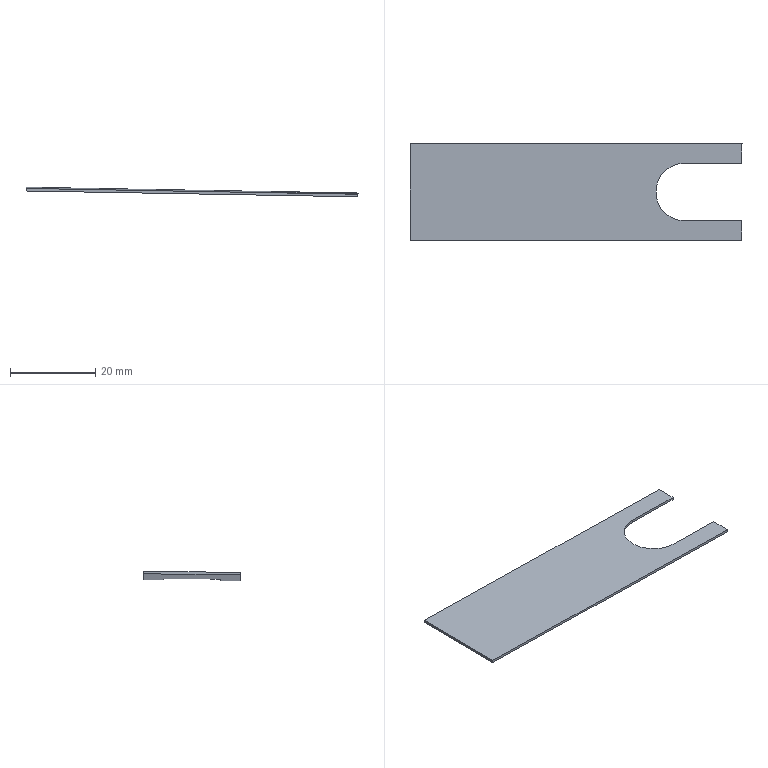Component | SolidWorks | 00-VacuumSuctionCupAssembly-1_02-TopCoverPlate-1 | 1 solid | 10 faces | box 78 x 22.66 x 2.25 mm | volume 908 mm3 | plane 9 | cylinder 1 | commonest cylinder face diameters 13.5 x1
build123d program:
from build123d import *

# Parameters (mm, degrees)
BOSS_EXTRUDE1_DEPTH = 2
SCALE1_SCALE        = 0.3


with BuildPart() as part:
    # Sketch1 → Boss-Extrude1 (new body)
    with BuildSketch(Plane(origin=(0, 2, 0), x_dir=(1, 0, 0), z_dir=(0, 1, 0))):
        with BuildLine():
            Line((45, -22.5), (0, -22.5))
            Line((0, -22.5), (0, -37.75))
            Line((0, -37.75), (260, -37.75))
            Line((260, -37.75), (260, 37.75))
            Line((260, 37.75), (0, 37.75))
            Line((0, 37.75), (0, 22.5))
            Line((0, 22.5), (45, 22.5))
            ThreePointArc((45, 22.5), (67.5, 0), (45, -22.5))
        make_face()
    extrude(amount=-BOSS_EXTRUDE1_DEPTH)


with BuildPart() as part_1:
    # Scale1: scaled about (146.519, 1, 0)
    add(part.part.scale(SCALE1_SCALE).moved(Location((102.564, 0.7, 0))))


solid = part_1.part

# Placed as in the assembly
solid = solid.moved(Location((174.24, 133.834, 29.789), (-89.279, 0.01259, -179)))
STEP:
#1=COLOUR_RGB('',0.7922,0.8196,0.9333);
#2=FILL_AREA_STYLE_COLOUR('',#1);
#3=FILL_AREA_STYLE('',(#2));
#4=SURFACE_STYLE_FILL_AREA(#3);
#5=SURFACE_SIDE_STYLE('',(#4));
#6=SURFACE_STYLE_USAGE(.BOTH.,#5);
#7=PRESENTATION_STYLE_ASSIGNMENT((#6));
#8=CARTESIAN_POINT('',(2.292,5.534,1.283));
#9=VERTEX_POINT('',#8);
#10=CARTESIAN_POINT('',(2.292,5.003,1.277));
#11=VERTEX_POINT('',#10);
#12=CARTESIAN_POINT('',(2.292,5.269,1.28));
#13=DIRECTION('',(0.01745,-0.01259,0.9998));
#14=DIRECTION('',(0.0002197,0.9999,0.01259));
#15=AXIS2_PLACEMENT_3D('',#12,#13,#14);
#16=CIRCLE('',#15,0.2657);
#17=EDGE_CURVE('',#9,#11,#16,.T.);
#18=ORIENTED_EDGE('',*,*,#17,.F.);
#19=CARTESIAN_POINT('',(2.292,5.534,1.307));
#20=VERTEX_POINT('',#19);
#21=CARTESIAN_POINT('',(2.292,5.534,1.307));
#22=DIRECTION('',(-0.01745,0.01259,-0.9998));
#23=VECTOR('',#22,39.37);
#24=LINE('',#21,#23);
#25=EDGE_CURVE('',#20,#9,#24,.T.);
#26=ORIENTED_EDGE('',*,*,#25,.F.);
#27=CARTESIAN_POINT('',(2.292,5.003,1.3));
#28=VERTEX_POINT('',#27);
#29=CARTESIAN_POINT('',(2.292,5.268,1.304));
#30=DIRECTION('',(0.01745,-0.01259,0.9998));
#31=DIRECTION('',(0.0002197,0.9999,0.01259));
#32=AXIS2_PLACEMENT_3D('',#29,#30,#31);
#33=CIRCLE('',#32,0.2657);
#34=EDGE_CURVE('',#20,#28,#33,.T.);
#35=ORIENTED_EDGE('',*,*,#34,.T.);
#36=CARTESIAN_POINT('',(2.292,5.003,1.3));
#37=DIRECTION('',(-0.01745,0.01259,-0.9998));
#38=VECTOR('',#37,39.37);
#39=LINE('',#36,#38);
#40=EDGE_CURVE('',#28,#11,#39,.T.);
#41=ORIENTED_EDGE('',*,*,#40,.T.);
#42=EDGE_LOOP('',(#18,#26,#35,#41));
#43=FACE_OUTER_BOUND('',#42,.T.);
#44=CARTESIAN_POINT('',(2.292,5.268,1.304));
#45=DIRECTION('',(-0.01745,0.01259,-0.9998));
#46=DIRECTION('',(-0.0002197,-0.9999,-0.01259));
#47=AXIS2_PLACEMENT_3D('',#44,#45,#46);
#48=CYLINDRICAL_SURFACE('',#47,0.2657);
#49=ADVANCED_FACE('',(#43),#48,.F.);
#50=CARTESIAN_POINT('',(2.823,5.534,1.274));
#51=VERTEX_POINT('',#50);
#52=CARTESIAN_POINT('',(2.823,5.534,1.274));
#53=DIRECTION('',(-0.9998,0.,0.01745));
#54=VECTOR('',#53,39.37);
#55=LINE('',#52,#54);
#56=EDGE_CURVE('',#51,#9,#55,.T.);
#57=ORIENTED_EDGE('',*,*,#56,.F.);
#58=CARTESIAN_POINT('',(2.823,5.534,1.298));
#59=VERTEX_POINT('',#58);
#60=CARTESIAN_POINT('',(2.823,5.534,1.298));
#61=DIRECTION('',(-0.01745,0.01259,-0.9998));
#62=VECTOR('',#61,39.37);
#63=LINE('',#60,#62);
#64=EDGE_CURVE('',#59,#51,#63,.T.);
#65=ORIENTED_EDGE('',*,*,#64,.F.);
#66=CARTESIAN_POINT('',(2.823,5.534,1.298));
#67=DIRECTION('',(-0.9998,0.,0.01745));
#68=VECTOR('',#67,39.37);
#69=LINE('',#66,#68);
#70=EDGE_CURVE('',#59,#20,#69,.T.);
#71=ORIENTED_EDGE('',*,*,#70,.T.);
#72=ORIENTED_EDGE('',*,*,#25,.T.);
#73=EDGE_LOOP('',(#57,#65,#71,#72));
#74=FACE_OUTER_BOUND('',#73,.T.);
#75=CARTESIAN_POINT('',(2.823,5.534,1.298));
#76=DIRECTION('',(-0.0002197,-0.9999,-0.01259));
#77=DIRECTION('',(-0.9998,0.,0.01745));
#78=AXIS2_PLACEMENT_3D('',#75,#76,#77);
#79=PLANE('',#78);
#80=ADVANCED_FACE('',(#74),#79,.T.);
#81=CARTESIAN_POINT('',(2.823,5.715,1.276));
#82=VERTEX_POINT('',#81);
#83=CARTESIAN_POINT('',(2.823,5.715,1.276));
#84=DIRECTION('',(-0.0002197,-0.9999,-0.01259));
#85=VECTOR('',#84,39.37);
#86=LINE('',#83,#85);
#87=EDGE_CURVE('',#82,#51,#86,.T.);
#88=ORIENTED_EDGE('',*,*,#87,.F.);
#89=CARTESIAN_POINT('',(2.824,5.714,1.3));
#90=VERTEX_POINT('',#89);
#91=CARTESIAN_POINT('',(2.824,5.714,1.3));
#92=DIRECTION('',(-0.01745,0.01259,-0.9998));
#93=VECTOR('',#92,39.37);
#94=LINE('',#91,#93);
#95=EDGE_CURVE('',#90,#82,#94,.T.);
#96=ORIENTED_EDGE('',*,*,#95,.F.);
#97=CARTESIAN_POINT('',(2.824,5.714,1.3));
#98=DIRECTION('',(-0.0002197,-0.9999,-0.01259));
#99=VECTOR('',#98,39.37);
#100=LINE('',#97,#99);
#101=EDGE_CURVE('',#90,#59,#100,.T.);
#102=ORIENTED_EDGE('',*,*,#101,.T.);
#103=ORIENTED_EDGE('',*,*,#64,.T.);
#104=EDGE_LOOP('',(#88,#96,#102,#103));
#105=FACE_OUTER_BOUND('',#104,.T.);
#106=CARTESIAN_POINT('',(2.824,5.714,1.3));
#107=DIRECTION('',(0.9998,-0.,-0.01745));
#108=DIRECTION('',(-0.0002197,-0.9999,-0.01259));
#109=AXIS2_PLACEMENT_3D('',#106,#107,#108);
#110=PLANE('',#109);
#111=ADVANCED_FACE('',(#105),#110,.T.);
#112=CARTESIAN_POINT('',(-0.2473,5.715,1.33));
#113=VERTEX_POINT('',#112);
#114=CARTESIAN_POINT('',(-0.2473,5.715,1.33));
#115=DIRECTION('',(0.9998,-0.,-0.01745));
#116=VECTOR('',#115,39.37);
#117=LINE('',#114,#116);
#118=EDGE_CURVE('',#113,#82,#117,.T.);
#119=ORIENTED_EDGE('',*,*,#118,.F.);
#120=CARTESIAN_POINT('',(-0.2469,5.714,1.354));
#121=VERTEX_POINT('',#120);
#122=CARTESIAN_POINT('',(-0.2469,5.714,1.354));
#123=DIRECTION('',(-0.01745,0.01259,-0.9998));
#124=VECTOR('',#123,39.37);
#125=LINE('',#122,#124);
#126=EDGE_CURVE('',#121,#113,#125,.T.);
#127=ORIENTED_EDGE('',*,*,#126,.F.);
#128=CARTESIAN_POINT('',(-0.2469,5.714,1.354));
#129=DIRECTION('',(0.9998,-0.,-0.01745));
#130=VECTOR('',#129,39.37);
#131=LINE('',#128,#130);
#132=EDGE_CURVE('',#121,#90,#131,.T.);
#133=ORIENTED_EDGE('',*,*,#132,.T.);
#134=ORIENTED_EDGE('',*,*,#95,.T.);
#135=EDGE_LOOP('',(#119,#127,#133,#134));
#136=FACE_OUTER_BOUND('',#135,.T.);
#137=CARTESIAN_POINT('',(-0.2469,5.714,1.354));
#138=DIRECTION('',(0.0002197,0.9999,0.01259));
#139=DIRECTION('',(0.9998,-0.,-0.01745));
#140=AXIS2_PLACEMENT_3D('',#137,#138,#139);
#141=PLANE('',#140);
#142=ADVANCED_FACE('',(#136),#141,.T.);
#143=CARTESIAN_POINT('',(-0.2475,4.823,1.319));
#144=VERTEX_POINT('',#143);
#145=CARTESIAN_POINT('',(-0.2475,4.823,1.319));
#146=DIRECTION('',(0.0002197,0.9999,0.01259));
#147=VECTOR('',#146,39.37);
#148=LINE('',#145,#147);
#149=EDGE_CURVE('',#144,#113,#148,.T.);
#150=ORIENTED_EDGE('',*,*,#149,.F.);
#151=CARTESIAN_POINT('',(-0.2471,4.823,1.342));
#152=VERTEX_POINT('',#151);
#153=CARTESIAN_POINT('',(-0.2471,4.823,1.342));
#154=DIRECTION('',(-0.01745,0.01259,-0.9998));
#155=VECTOR('',#154,39.37);
#156=LINE('',#153,#155);
#157=EDGE_CURVE('',#152,#144,#156,.T.);
#158=ORIENTED_EDGE('',*,*,#157,.F.);
#159=CARTESIAN_POINT('',(-0.2471,4.823,1.342));
#160=DIRECTION('',(0.0002197,0.9999,0.01259));
#161=VECTOR('',#160,39.37);
#162=LINE('',#159,#161);
#163=EDGE_CURVE('',#152,#121,#162,.T.);
#164=ORIENTED_EDGE('',*,*,#163,.T.);
#165=ORIENTED_EDGE('',*,*,#126,.T.);
#166=EDGE_LOOP('',(#150,#158,#164,#165));
#167=FACE_OUTER_BOUND('',#166,.T.);
#168=CARTESIAN_POINT('',(-0.2471,4.823,1.342));
#169=DIRECTION('',(-0.9998,0.,0.01745));
#170=DIRECTION('',(0.0002197,0.9999,0.01259));
#171=AXIS2_PLACEMENT_3D('',#168,#169,#170);
#172=PLANE('',#171);
#173=ADVANCED_FACE('',(#167),#172,.T.);
#174=CARTESIAN_POINT('',(2.823,4.823,1.265));
#175=VERTEX_POINT('',#174);
#176=CARTESIAN_POINT('',(2.823,4.823,1.265));
#177=DIRECTION('',(-0.9998,0.,0.01745));
#178=VECTOR('',#177,39.37);
#179=LINE('',#176,#178);
#180=EDGE_CURVE('',#175,#144,#179,.T.);
#181=ORIENTED_EDGE('',*,*,#180,.F.);
#182=CARTESIAN_POINT('',(2.823,4.823,1.289));
#183=VERTEX_POINT('',#182);
#184=CARTESIAN_POINT('',(2.823,4.823,1.289));
#185=DIRECTION('',(-0.01745,0.01259,-0.9998));
#186=VECTOR('',#185,39.37);
#187=LINE('',#184,#186);
#188=EDGE_CURVE('',#183,#175,#187,.T.);
#189=ORIENTED_EDGE('',*,*,#188,.F.);
#190=CARTESIAN_POINT('',(2.823,4.823,1.289));
#191=DIRECTION('',(-0.9998,0.,0.01745));
#192=VECTOR('',#191,39.37);
#193=LINE('',#190,#192);
#194=EDGE_CURVE('',#183,#152,#193,.T.);
#195=ORIENTED_EDGE('',*,*,#194,.T.);
#196=ORIENTED_EDGE('',*,*,#157,.T.);
#197=EDGE_LOOP('',(#181,#189,#195,#196));
#198=FACE_OUTER_BOUND('',#197,.T.);
#199=CARTESIAN_POINT('',(2.823,4.823,1.289));
#200=DIRECTION('',(-0.0002197,-0.9999,-0.01259));
#201=DIRECTION('',(-0.9998,0.,0.01745));
#202=AXIS2_PLACEMENT_3D('',#199,#200,#201);
#203=PLANE('',#202);
#204=ADVANCED_FACE('',(#198),#203,.T.);
#205=CARTESIAN_POINT('',(2.823,5.003,1.267));
#206=VERTEX_POINT('',#205);
#207=CARTESIAN_POINT('',(2.823,5.003,1.267));
#208=DIRECTION('',(-0.0002197,-0.9999,-0.01259));
#209=VECTOR('',#208,39.37);
#210=LINE('',#207,#209);
#211=EDGE_CURVE('',#206,#175,#210,.T.);
#212=ORIENTED_EDGE('',*,*,#211,.F.);
#213=CARTESIAN_POINT('',(2.823,5.003,1.291));
#214=VERTEX_POINT('',#213);
#215=CARTESIAN_POINT('',(2.823,5.003,1.291));
#216=DIRECTION('',(-0.01745,0.01259,-0.9998));
#217=VECTOR('',#216,39.37);
#218=LINE('',#215,#217);
#219=EDGE_CURVE('',#214,#206,#218,.T.);
#220=ORIENTED_EDGE('',*,*,#219,.F.);
#221=CARTESIAN_POINT('',(2.823,5.003,1.291));
#222=DIRECTION('',(-0.0002197,-0.9999,-0.01259));
#223=VECTOR('',#222,39.37);
#224=LINE('',#221,#223);
#225=EDGE_CURVE('',#214,#183,#224,.T.);
#226=ORIENTED_EDGE('',*,*,#225,.T.);
#227=ORIENTED_EDGE('',*,*,#188,.T.);
#228=EDGE_LOOP('',(#212,#220,#226,#227));
#229=FACE_OUTER_BOUND('',#228,.T.);
#230=CARTESIAN_POINT('',(2.823,5.003,1.291));
#231=DIRECTION('',(0.9998,-0.,-0.01745));
#232=DIRECTION('',(-0.0002197,-0.9999,-0.01259));
#233=AXIS2_PLACEMENT_3D('',#230,#231,#232);
#234=PLANE('',#233);
#235=ADVANCED_FACE('',(#229),#234,.T.);
#236=CARTESIAN_POINT('',(2.292,5.003,1.277));
#237=DIRECTION('',(0.9998,-0.,-0.01745));
#238=VECTOR('',#237,39.37);
#239=LINE('',#236,#238);
#240=EDGE_CURVE('',#11,#206,#239,.T.);
#241=ORIENTED_EDGE('',*,*,#240,.F.);
#242=ORIENTED_EDGE('',*,*,#40,.F.);
#243=CARTESIAN_POINT('',(2.292,5.003,1.3));
#244=DIRECTION('',(0.9998,-0.,-0.01745));
#245=VECTOR('',#244,39.37);
#246=LINE('',#243,#245);
#247=EDGE_CURVE('',#28,#214,#246,.T.);
#248=ORIENTED_EDGE('',*,*,#247,.T.);
#249=ORIENTED_EDGE('',*,*,#219,.T.);
#250=EDGE_LOOP('',(#241,#242,#248,#249));
#251=FACE_OUTER_BOUND('',#250,.T.);
#252=CARTESIAN_POINT('',(2.292,5.003,1.3));
#253=DIRECTION('',(0.0002197,0.9999,0.01259));
#254=DIRECTION('',(0.9998,-0.,-0.01745));
#255=AXIS2_PLACEMENT_3D('',#252,#253,#254);
#256=PLANE('',#255);
#257=ADVANCED_FACE('',(#251),#256,.T.);
#258=ORIENTED_EDGE('',*,*,#34,.F.);
#259=ORIENTED_EDGE('',*,*,#70,.F.);
#260=ORIENTED_EDGE('',*,*,#101,.F.);
#261=ORIENTED_EDGE('',*,*,#132,.F.);
#262=ORIENTED_EDGE('',*,*,#163,.F.);
#263=ORIENTED_EDGE('',*,*,#194,.F.);
#264=ORIENTED_EDGE('',*,*,#225,.F.);
#265=ORIENTED_EDGE('',*,*,#247,.F.);
#266=EDGE_LOOP('',(#258,#259,#260,#261,#262,#263,#264,#265));
#267=FACE_OUTER_BOUND('',#266,.T.);
#268=CARTESIAN_POINT('',(2.292,5.268,1.304));
#269=DIRECTION('',(0.01745,-0.01259,0.9998));
#270=DIRECTION('',(0.0002197,0.9999,0.01259));
#271=AXIS2_PLACEMENT_3D('',#268,#269,#270);
#272=PLANE('',#271);
#273=ADVANCED_FACE('',(#267),#272,.T.);
#274=ORIENTED_EDGE('',*,*,#17,.T.);
#275=ORIENTED_EDGE('',*,*,#240,.T.);
#276=ORIENTED_EDGE('',*,*,#211,.T.);
#277=ORIENTED_EDGE('',*,*,#180,.T.);
#278=ORIENTED_EDGE('',*,*,#149,.T.);
#279=ORIENTED_EDGE('',*,*,#118,.T.);
#280=ORIENTED_EDGE('',*,*,#87,.T.);
#281=ORIENTED_EDGE('',*,*,#56,.T.);
#282=EDGE_LOOP('',(#274,#275,#276,#277,#278,#279,#280,#281));
#283=FACE_OUTER_BOUND('',#282,.T.);
#284=CARTESIAN_POINT('',(2.292,5.269,1.28));
#285=DIRECTION('',(0.01745,-0.01259,0.9998));
#286=DIRECTION('',(0.0002197,0.9999,0.01259));
#287=AXIS2_PLACEMENT_3D('',#284,#285,#286);
#288=PLANE('',#287);
#289=ADVANCED_FACE('',(#283),#288,.F.);
#290=CLOSED_SHELL('',(#49,#80,#111,#142,#173,#204,#235,#257,#273,#289));
#291=MANIFOLD_SOLID_BREP('',#290);
#292=STYLED_ITEM('',(#7),#291);
#293=PRESENTATION_LAYER_ASSIGNMENT('','',(#292));
#294=CARTESIAN_POINT('',(0.,0.,0.));
#295=DIRECTION('',(0.,0.,1.));
#296=DIRECTION('',(1.,0.,0.));
#297=AXIS2_PLACEMENT_3D('',#294,#295,#296);
#298=(LENGTH_UNIT()NAMED_UNIT(*)SI_UNIT($,.METRE.));
#299=LENGTH_MEASURE_WITH_UNIT(LENGTH_MEASURE(0.0254),#298);
#300=DIMENSIONAL_EXPONENTS(1.,0.,0.,0.,0.,0.,0.);
#301=(CONVERSION_BASED_UNIT('',#299)LENGTH_UNIT()NAMED_UNIT(#300));
#302=UNCERTAINTY_MEASURE_WITH_UNIT(LENGTH_MEASURE(0.00001),#301,'','');
#303=(NAMED_UNIT(*)PLANE_ANGLE_UNIT()SI_UNIT($,.RADIAN.));
#304=(NAMED_UNIT(*)SI_UNIT($,.STERADIAN.)SOLID_ANGLE_UNIT());
#305=(GEOMETRIC_REPRESENTATION_CONTEXT(3)GLOBAL_UNCERTAINTY_ASSIGNED_CONTEXT((#302))GLOBAL_UNIT_ASSIGNED_CONTEXT((#301,#303,#304))REPRESENTATION_CONTEXT('',''));
#306=ADVANCED_BREP_SHAPE_REPRESENTATION('',(#291,#297),#305);
#307=(LENGTH_UNIT()NAMED_UNIT(*)SI_UNIT($,.METRE.));
#308=LENGTH_MEASURE_WITH_UNIT(LENGTH_MEASURE(0.0254),#307);
#309=DIMENSIONAL_EXPONENTS(1.,0.,0.,0.,0.,0.,0.);
#310=(CONVERSION_BASED_UNIT('',#308)LENGTH_UNIT()NAMED_UNIT(#309));
#311=UNCERTAINTY_MEASURE_WITH_UNIT(LENGTH_MEASURE(0.00001),#310,'','');
#312=(NAMED_UNIT(*)PLANE_ANGLE_UNIT()SI_UNIT($,.RADIAN.));
#313=(NAMED_UNIT(*)SI_UNIT($,.STERADIAN.)SOLID_ANGLE_UNIT());
#314=(GEOMETRIC_REPRESENTATION_CONTEXT(3)GLOBAL_UNCERTAINTY_ASSIGNED_CONTEXT((#311))GLOBAL_UNIT_ASSIGNED_CONTEXT((#310,#312,#313))REPRESENTATION_CONTEXT('',''));
#315=MECHANICAL_DESIGN_GEOMETRIC_PRESENTATION_REPRESENTATION('',(#292),#314);